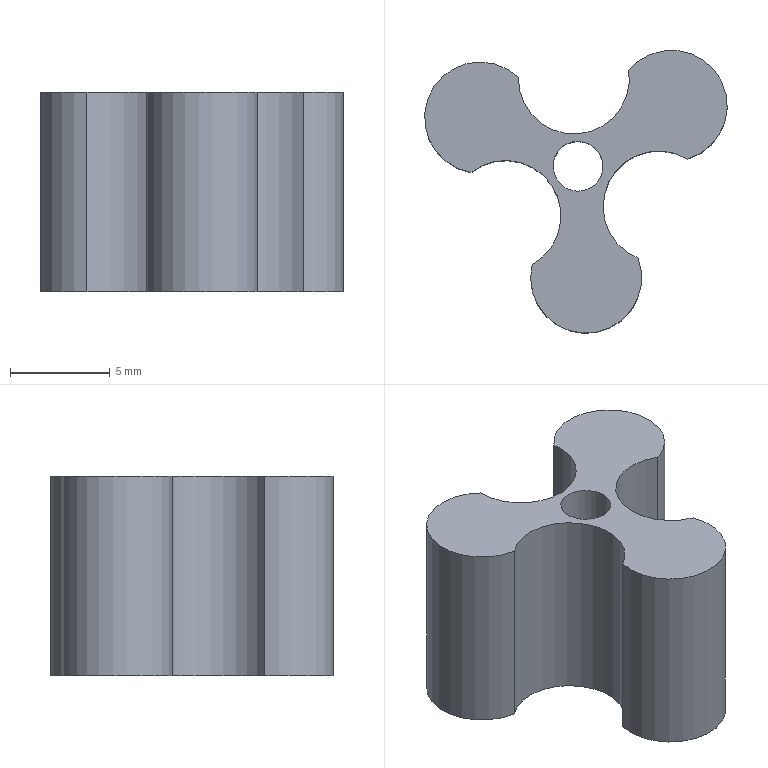Component | NX | ROTOR_2 | 1 solid | 9 faces | box 15.17 x 14.18 x 10 mm | volume 814 mm3 | cylinder 7 | plane 2 | commonest cylinder face diameters 5.568 x6 2.5 x1
STEP:
#1=CARTESIAN_POINT('',(0.,0.,0.));
#2=DIRECTION('',(0.,0.,1.));
#3=DIRECTION('',(1.,0.,0.));
#4=AXIS2_PLACEMENT_3D('',#1,#2,#3);
#5=CARTESIAN_POINT('',(8.277,-4.62,-5.));
#6=VERTEX_POINT('',#5);
#7=CARTESIAN_POINT('',(2.964,-4.947,-5.));
#8=VERTEX_POINT('',#7);
#9=CARTESIAN_POINT('',(5.671,-5.598,-5.));
#10=DIRECTION('',(0.,0.,-1.));
#11=DIRECTION('',(-0.06144,0.9981,0.));
#12=AXIS2_PLACEMENT_3D('',#9,#10,#11);
#13=CIRCLE('',#12,2.784);
#14=CARTESIAN_POINT('',(3.648,-4.052,-5.));
#15=DIRECTION('',(0.,0.,-1.));
#16=DIRECTION('',(-0.8337,-0.5523,0.));
#17=AXIS2_PLACEMENT_3D('',#14,#15,#16);
#18=PLANE('',#17);
#19=CARTESIAN_POINT('',(-0.833,-2.406));
#20=DIRECTION('',(-0.5,0.866));
#21=AXIS2_PLACEMENT_2D('',#19,#20);
#22=CIRCLE('',#21,2.784);
#23=(GEOMETRIC_REPRESENTATION_CONTEXT(2)PARAMETRIC_REPRESENTATION_CONTEXT()REPRESENTATION_CONTEXT('',''));
#24=DEFINITIONAL_REPRESENTATION('',(#22),#23);
#25=PCURVE('',#18,#24);
#26=CARTESIAN_POINT('',(5.671,-5.598,-5.));
#27=DIRECTION('',(0.,0.,1.));
#28=DIRECTION('',(0.8337,0.5523,0.));
#29=AXIS2_PLACEMENT_3D('',#26,#27,#28);
#30=CYLINDRICAL_SURFACE('',#29,2.784);
#31=CARTESIAN_POINT('',(7.33,0.));
#32=DIRECTION('',(-1.,0.));
#33=VECTOR('',#32,1.);
#34=LINE('',#31,#33);
#35=(GEOMETRIC_REPRESENTATION_CONTEXT(2)PARAMETRIC_REPRESENTATION_CONTEXT()REPRESENTATION_CONTEXT('',''));
#36=DEFINITIONAL_REPRESENTATION('',(#34),#35);
#37=PCURVE('',#30,#36);
#38=SURFACE_CURVE('',#13,(#25,#37),.PCURVE_S1.);
#39=EDGE_CURVE('',#6,#8,#38,.T.);
#40=ORIENTED_EDGE('',*,*,#39,.T.);
#41=CARTESIAN_POINT('',(-0.1006,-0.3217,-5.));
#42=VERTEX_POINT('',#41);
#43=CARTESIAN_POINT('',(1.625,-2.507,-5.));
#44=DIRECTION('',(0.,0.,1.));
#45=DIRECTION('',(-0.06144,0.9981,0.));
#46=AXIS2_PLACEMENT_3D('',#43,#44,#45);
#47=CIRCLE('',#46,2.784);
#48=CARTESIAN_POINT('',(-0.559,4.817));
#49=CARTESIAN_POINT('',(3.617,7.228));
#50=CARTESIAN_POINT('',(3.617,2.406));
#51=CARTESIAN_POINT('',(3.617,-2.416));
#52=CARTESIAN_POINT('',(-0.559,-0.005196));
#53=CARTESIAN_POINT('',(-4.735,2.406));
#54=CARTESIAN_POINT('',(-0.559,4.817));
#55=(BOUNDED_CURVE()B_SPLINE_CURVE(2,(#48,#49,#50,#51,#52,#53,#54),.UNSPECIFIED.,.T.,.F.)B_SPLINE_CURVE_WITH_KNOTS((1,2,2,2,2,1),(-2.094,0.,2.094,4.189,6.283,8.378),.UNSPECIFIED.)CURVE()GEOMETRIC_REPRESENTATION_ITEM()RATIONAL_B_SPLINE_CURVE((1.,0.5,1.,0.5,1.,0.5,1.))REPRESENTATION_ITEM(''));
#56=(GEOMETRIC_REPRESENTATION_CONTEXT(2)PARAMETRIC_REPRESENTATION_CONTEXT()REPRESENTATION_CONTEXT('',''));
#57=DEFINITIONAL_REPRESENTATION('',(#55),#56);
#58=PCURVE('',#18,#57);
#59=CARTESIAN_POINT('',(1.625,-2.507,-5.));
#60=DIRECTION('',(0.,0.,1.));
#61=DIRECTION('',(0.8337,0.5523,0.));
#62=AXIS2_PLACEMENT_3D('',#59,#60,#61);
#63=CYLINDRICAL_SURFACE('',#62,2.784);
#64=CARTESIAN_POINT('',(-5.236,0.));
#65=DIRECTION('',(1.,0.));
#66=VECTOR('',#65,1.);
#67=LINE('',#64,#66);
#68=(GEOMETRIC_REPRESENTATION_CONTEXT(2)PARAMETRIC_REPRESENTATION_CONTEXT()REPRESENTATION_CONTEXT('',''));
#69=DEFINITIONAL_REPRESENTATION('',(#67),#68);
#70=PCURVE('',#63,#69);
#71=SURFACE_CURVE('',#47,(#58,#70),.PCURVE_S1.);
#72=EDGE_CURVE('',#8,#42,#71,.T.);
#73=ORIENTED_EDGE('',*,*,#72,.T.);
#74=CARTESIAN_POINT('',(2.273,4.444,-5.));
#75=VERTEX_POINT('',#74);
#76=CARTESIAN_POINT('',(0.3561,2.425,-5.));
#77=DIRECTION('',(0.,0.,-1.));
#78=DIRECTION('',(-0.8337,-0.5523,0.));
#79=AXIS2_PLACEMENT_3D('',#76,#77,#78);
#80=CIRCLE('',#79,2.784);
#81=CARTESIAN_POINT('',(-0.833,7.217));
#82=DIRECTION('',(1.,0.));
#83=AXIS2_PLACEMENT_2D('',#81,#82);
#84=CIRCLE('',#83,2.784);
#85=(GEOMETRIC_REPRESENTATION_CONTEXT(2)PARAMETRIC_REPRESENTATION_CONTEXT()REPRESENTATION_CONTEXT('',''));
#86=DEFINITIONAL_REPRESENTATION('',(#84),#85);
#87=PCURVE('',#18,#86);
#88=CARTESIAN_POINT('',(0.3561,2.425,-5.));
#89=DIRECTION('',(0.,0.,1.));
#90=DIRECTION('',(0.8337,0.5523,0.));
#91=AXIS2_PLACEMENT_3D('',#88,#89,#90);
#92=CYLINDRICAL_SURFACE('',#91,2.784);
#93=CARTESIAN_POINT('',(9.425,0.));
#94=DIRECTION('',(-1.,0.));
#95=VECTOR('',#94,1.);
#96=LINE('',#93,#95);
#97=(GEOMETRIC_REPRESENTATION_CONTEXT(2)PARAMETRIC_REPRESENTATION_CONTEXT()REPRESENTATION_CONTEXT('',''));
#98=DEFINITIONAL_REPRESENTATION('',(#96),#97);
#99=PCURVE('',#92,#98);
#100=SURFACE_CURVE('',#80,(#87,#99),.PCURVE_S1.);
#101=EDGE_CURVE('',#42,#75,#100,.T.);
#102=ORIENTED_EDGE('',*,*,#101,.T.);
#103=CARTESIAN_POINT('',(7.811,4.785,-5.));
#104=VERTEX_POINT('',#103);
#105=CARTESIAN_POINT('',(5.056,4.383,-5.));
#106=DIRECTION('',(0.,0.,1.));
#107=DIRECTION('',(-0.06144,0.9981,0.));
#108=AXIS2_PLACEMENT_3D('',#105,#106,#107);
#109=CIRCLE('',#108,2.784);
#110=CARTESIAN_POINT('',(-7.225,8.665));
#111=CARTESIAN_POINT('',(-3.049,11.076));
#112=CARTESIAN_POINT('',(-3.049,6.254));
#113=CARTESIAN_POINT('',(-3.049,1.432));
#114=CARTESIAN_POINT('',(-7.225,3.843));
#115=CARTESIAN_POINT('',(-11.401,6.254));
#116=CARTESIAN_POINT('',(-7.225,8.665));
#117=(BOUNDED_CURVE()B_SPLINE_CURVE(2,(#110,#111,#112,#113,#114,#115,#116),.UNSPECIFIED.,.T.,.F.)B_SPLINE_CURVE_WITH_KNOTS((1,2,2,2,2,1),(-2.094,0.,2.094,4.189,6.283,8.378),.UNSPECIFIED.)CURVE()GEOMETRIC_REPRESENTATION_ITEM()RATIONAL_B_SPLINE_CURVE((1.,0.5,1.,0.5,1.,0.5,1.))REPRESENTATION_ITEM(''));
#118=(GEOMETRIC_REPRESENTATION_CONTEXT(2)PARAMETRIC_REPRESENTATION_CONTEXT()REPRESENTATION_CONTEXT('',''));
#119=DEFINITIONAL_REPRESENTATION('',(#117),#118);
#120=PCURVE('',#18,#119);
#121=CARTESIAN_POINT('',(5.056,4.383,-5.));
#122=DIRECTION('',(0.,0.,1.));
#123=DIRECTION('',(0.8337,0.5523,0.));
#124=AXIS2_PLACEMENT_3D('',#121,#122,#123);
#125=CYLINDRICAL_SURFACE('',#124,2.784);
#126=CARTESIAN_POINT('',(1.047,0.));
#127=DIRECTION('',(1.,0.));
#128=VECTOR('',#127,1.);
#129=LINE('',#126,#128);
#130=(GEOMETRIC_REPRESENTATION_CONTEXT(2)PARAMETRIC_REPRESENTATION_CONTEXT()REPRESENTATION_CONTEXT('',''));
#131=DEFINITIONAL_REPRESENTATION('',(#129),#130);
#132=PCURVE('',#125,#131);
#133=SURFACE_CURVE('',#109,(#120,#132),.PCURVE_S1.);
#134=EDGE_CURVE('',#75,#104,#133,.T.);
#135=ORIENTED_EDGE('',*,*,#134,.T.);
#136=CARTESIAN_POINT('',(10.751,0.3464,-5.));
#137=VERTEX_POINT('',#136);
#138=CARTESIAN_POINT('',(9.961,3.016,-5.));
#139=DIRECTION('',(0.,0.,-1.));
#140=DIRECTION('',(-0.8337,-0.5523,0.));
#141=AXIS2_PLACEMENT_3D('',#138,#139,#140);
#142=CIRCLE('',#141,2.784);
#143=CARTESIAN_POINT('',(-9.167,2.406));
#144=DIRECTION('',(1.,0.));
#145=AXIS2_PLACEMENT_2D('',#143,#144);
#146=CIRCLE('',#145,2.784);
#147=(GEOMETRIC_REPRESENTATION_CONTEXT(2)PARAMETRIC_REPRESENTATION_CONTEXT()REPRESENTATION_CONTEXT('',''));
#148=DEFINITIONAL_REPRESENTATION('',(#146),#147);
#149=PCURVE('',#18,#148);
#150=CARTESIAN_POINT('',(9.961,3.016,-5.));
#151=DIRECTION('',(0.,0.,1.));
#152=DIRECTION('',(0.8337,0.5523,0.));
#153=AXIS2_PLACEMENT_3D('',#150,#151,#152);
#154=CYLINDRICAL_SURFACE('',#153,2.784);
#155=CARTESIAN_POINT('',(9.425,0.));
#156=DIRECTION('',(-1.,0.));
#157=VECTOR('',#156,1.);
#158=LINE('',#155,#157);
#159=(GEOMETRIC_REPRESENTATION_CONTEXT(2)PARAMETRIC_REPRESENTATION_CONTEXT()REPRESENTATION_CONTEXT('',''));
#160=DEFINITIONAL_REPRESENTATION('',(#158),#159);
#161=PCURVE('',#154,#160);
#162=SURFACE_CURVE('',#142,(#149,#161),.PCURVE_S1.);
#163=EDGE_CURVE('',#104,#137,#162,.T.);
#164=ORIENTED_EDGE('',*,*,#163,.T.);
#165=CARTESIAN_POINT('',(9.307,-2.034,-5.));
#166=DIRECTION('',(0.,0.,1.));
#167=DIRECTION('',(-0.06144,0.9981,0.));
#168=AXIS2_PLACEMENT_3D('',#165,#166,#167);
#169=CIRCLE('',#168,2.784);
#170=CARTESIAN_POINT('',(-7.225,0.9682));
#171=CARTESIAN_POINT('',(-3.049,3.379));
#172=CARTESIAN_POINT('',(-3.049,-1.443));
#173=CARTESIAN_POINT('',(-3.049,-6.265));
#174=CARTESIAN_POINT('',(-7.225,-3.854));
#175=CARTESIAN_POINT('',(-11.401,-1.443));
#176=CARTESIAN_POINT('',(-7.225,0.9682));
#177=(BOUNDED_CURVE()B_SPLINE_CURVE(2,(#170,#171,#172,#173,#174,#175,#176),.UNSPECIFIED.,.T.,.F.)B_SPLINE_CURVE_WITH_KNOTS((1,2,2,2,2,1),(-2.094,0.,2.094,4.189,6.283,8.378),.UNSPECIFIED.)CURVE()GEOMETRIC_REPRESENTATION_ITEM()RATIONAL_B_SPLINE_CURVE((1.,0.5,1.,0.5,1.,0.5,1.))REPRESENTATION_ITEM(''));
#178=(GEOMETRIC_REPRESENTATION_CONTEXT(2)PARAMETRIC_REPRESENTATION_CONTEXT()REPRESENTATION_CONTEXT('',''));
#179=DEFINITIONAL_REPRESENTATION('',(#177),#178);
#180=PCURVE('',#18,#179);
#181=CARTESIAN_POINT('',(9.307,-2.034,-5.));
#182=DIRECTION('',(0.,0.,1.));
#183=DIRECTION('',(0.8337,0.5523,0.));
#184=AXIS2_PLACEMENT_3D('',#181,#182,#183);
#185=CYLINDRICAL_SURFACE('',#184,2.784);
#186=CARTESIAN_POINT('',(-5.236,0.));
#187=DIRECTION('',(1.,0.));
#188=VECTOR('',#187,1.);
#189=LINE('',#186,#188);
#190=(GEOMETRIC_REPRESENTATION_CONTEXT(2)PARAMETRIC_REPRESENTATION_CONTEXT()REPRESENTATION_CONTEXT('',''));
#191=DEFINITIONAL_REPRESENTATION('',(#189),#190);
#192=PCURVE('',#185,#191);
#193=SURFACE_CURVE('',#169,(#180,#192),.PCURVE_S1.);
#194=EDGE_CURVE('',#137,#6,#193,.T.);
#195=ORIENTED_EDGE('',*,*,#194,.T.);
#196=EDGE_LOOP('',(#40,#73,#102,#135,#164,#195));
#197=FACE_BOUND('',#196,.T.);
#198=CARTESIAN_POINT('',(4.224,-0.7066,-5.));
#199=VERTEX_POINT('',#198);
#200=CARTESIAN_POINT('',(5.266,-0.01624,-5.));
#201=DIRECTION('',(0.,0.,1.));
#202=DIRECTION('',(-0.8337,-0.5523,0.));
#203=AXIS2_PLACEMENT_3D('',#200,#201,#202);
#204=CIRCLE('',#203,1.25);
#205=CARTESIAN_POINT('',(-2.328,2.471));
#206=CARTESIAN_POINT('',(-2.328,0.3058));
#207=CARTESIAN_POINT('',(-4.203,1.388));
#208=CARTESIAN_POINT('',(-6.078,2.471));
#209=CARTESIAN_POINT('',(-4.203,3.553));
#210=CARTESIAN_POINT('',(-2.328,4.636));
#211=CARTESIAN_POINT('',(-2.328,2.471));
#212=(BOUNDED_CURVE()B_SPLINE_CURVE(2,(#205,#206,#207,#208,#209,#210,#211),.UNSPECIFIED.,.T.,.F.)B_SPLINE_CURVE_WITH_KNOTS((1,2,2,2,2,1),(-2.094,0.,2.094,4.189,6.283,8.378),.UNSPECIFIED.)CURVE()GEOMETRIC_REPRESENTATION_ITEM()RATIONAL_B_SPLINE_CURVE((1.,0.5,1.,0.5,1.,0.5,1.))REPRESENTATION_ITEM(''));
#213=(GEOMETRIC_REPRESENTATION_CONTEXT(2)PARAMETRIC_REPRESENTATION_CONTEXT()REPRESENTATION_CONTEXT('',''));
#214=DEFINITIONAL_REPRESENTATION('',(#212),#213);
#215=PCURVE('',#18,#214);
#216=CARTESIAN_POINT('',(5.266,-0.01624,-7.));
#217=DIRECTION('',(0.,0.,1.));
#218=DIRECTION('',(0.8337,0.5523,0.));
#219=AXIS2_PLACEMENT_3D('',#216,#217,#218);
#220=CYLINDRICAL_SURFACE('',#219,1.25);
#221=CARTESIAN_POINT('',(3.142,2.));
#222=DIRECTION('',(1.,0.));
#223=VECTOR('',#222,1.);
#224=LINE('',#221,#223);
#225=(GEOMETRIC_REPRESENTATION_CONTEXT(2)PARAMETRIC_REPRESENTATION_CONTEXT()REPRESENTATION_CONTEXT('',''));
#226=DEFINITIONAL_REPRESENTATION('',(#224),#225);
#227=PCURVE('',#220,#226);
#228=SURFACE_CURVE('',#204,(#215,#227),.PCURVE_S1.);
#229=EDGE_CURVE('',#199,#199,#228,.T.);
#230=ORIENTED_EDGE('',*,*,#229,.T.);
#231=EDGE_LOOP('',(#230));
#232=FACE_BOUND('',#231,.T.);
#233=ADVANCED_FACE('',(#197,#232),#18,.T.);
#234=CARTESIAN_POINT('',(2.964,-4.947,5.));
#235=VERTEX_POINT('',#234);
#236=CARTESIAN_POINT('',(-0.1006,-0.3217,5.));
#237=VERTEX_POINT('',#236);
#238=CARTESIAN_POINT('',(1.625,-2.507,5.));
#239=DIRECTION('',(0.,0.,1.));
#240=DIRECTION('',(-0.8337,-0.5523,0.));
#241=AXIS2_PLACEMENT_3D('',#238,#239,#240);
#242=CIRCLE('',#241,2.784);
#243=CARTESIAN_POINT('',(3.648,-4.052,5.));
#244=DIRECTION('',(0.,0.,-1.));
#245=DIRECTION('',(-0.8337,-0.5523,0.));
#246=AXIS2_PLACEMENT_3D('',#243,#244,#245);
#247=PLANE('',#246);
#248=CARTESIAN_POINT('',(3.617,2.406));
#249=CARTESIAN_POINT('',(3.617,-2.416));
#250=CARTESIAN_POINT('',(-0.559,-0.005196));
#251=CARTESIAN_POINT('',(-4.735,2.406));
#252=CARTESIAN_POINT('',(-0.559,4.817));
#253=CARTESIAN_POINT('',(3.617,7.228));
#254=CARTESIAN_POINT('',(3.617,2.406));
#255=(BOUNDED_CURVE()B_SPLINE_CURVE(2,(#248,#249,#250,#251,#252,#253,#254),.UNSPECIFIED.,.T.,.F.)B_SPLINE_CURVE_WITH_KNOTS((1,2,2,2,2,1),(-2.094,0.,2.094,4.189,6.283,8.378),.UNSPECIFIED.)CURVE()GEOMETRIC_REPRESENTATION_ITEM()RATIONAL_B_SPLINE_CURVE((1.,0.5,1.,0.5,1.,0.5,1.))REPRESENTATION_ITEM(''));
#256=(GEOMETRIC_REPRESENTATION_CONTEXT(2)PARAMETRIC_REPRESENTATION_CONTEXT()REPRESENTATION_CONTEXT('',''));
#257=DEFINITIONAL_REPRESENTATION('',(#255),#256);
#258=PCURVE('',#247,#257);
#259=CARTESIAN_POINT('',(-3.142,10.));
#260=DIRECTION('',(1.,0.));
#261=VECTOR('',#260,1.);
#262=LINE('',#259,#261);
#263=(GEOMETRIC_REPRESENTATION_CONTEXT(2)PARAMETRIC_REPRESENTATION_CONTEXT()REPRESENTATION_CONTEXT('',''));
#264=DEFINITIONAL_REPRESENTATION('',(#262),#263);
#265=PCURVE('',#63,#264);
#266=SURFACE_CURVE('',#242,(#258,#265),.PCURVE_S1.);
#267=EDGE_CURVE('',#235,#237,#266,.T.);
#268=ORIENTED_EDGE('',*,*,#267,.F.);
#269=CARTESIAN_POINT('',(8.277,-4.62,5.));
#270=VERTEX_POINT('',#269);
#271=CARTESIAN_POINT('',(5.671,-5.598,5.));
#272=DIRECTION('',(0.,0.,-1.));
#273=DIRECTION('',(-0.8337,-0.5523,0.));
#274=AXIS2_PLACEMENT_3D('',#271,#272,#273);
#275=CIRCLE('',#274,2.784);
#276=CARTESIAN_POINT('',(-0.833,-2.406));
#277=DIRECTION('',(1.,0.));
#278=AXIS2_PLACEMENT_2D('',#276,#277);
#279=CIRCLE('',#278,2.784);
#280=(GEOMETRIC_REPRESENTATION_CONTEXT(2)PARAMETRIC_REPRESENTATION_CONTEXT()REPRESENTATION_CONTEXT('',''));
#281=DEFINITIONAL_REPRESENTATION('',(#279),#280);
#282=PCURVE('',#247,#281);
#283=CARTESIAN_POINT('',(9.425,10.));
#284=DIRECTION('',(-1.,0.));
#285=VECTOR('',#284,1.);
#286=LINE('',#283,#285);
#287=(GEOMETRIC_REPRESENTATION_CONTEXT(2)PARAMETRIC_REPRESENTATION_CONTEXT()REPRESENTATION_CONTEXT('',''));
#288=DEFINITIONAL_REPRESENTATION('',(#286),#287);
#289=PCURVE('',#30,#288);
#290=SURFACE_CURVE('',#275,(#282,#289),.PCURVE_S1.);
#291=EDGE_CURVE('',#270,#235,#290,.T.);
#292=ORIENTED_EDGE('',*,*,#291,.F.);
#293=CARTESIAN_POINT('',(10.751,0.3464,5.));
#294=VERTEX_POINT('',#293);
#295=CARTESIAN_POINT('',(9.307,-2.034,5.));
#296=DIRECTION('',(0.,0.,1.));
#297=DIRECTION('',(-0.8337,-0.5523,0.));
#298=AXIS2_PLACEMENT_3D('',#295,#296,#297);
#299=CIRCLE('',#298,2.784);
#300=CARTESIAN_POINT('',(-3.049,-1.443));
#301=CARTESIAN_POINT('',(-3.049,-6.265));
#302=CARTESIAN_POINT('',(-7.225,-3.854));
#303=CARTESIAN_POINT('',(-11.401,-1.443));
#304=CARTESIAN_POINT('',(-7.225,0.9682));
#305=CARTESIAN_POINT('',(-3.049,3.379));
#306=CARTESIAN_POINT('',(-3.049,-1.443));
#307=(BOUNDED_CURVE()B_SPLINE_CURVE(2,(#300,#301,#302,#303,#304,#305,#306),.UNSPECIFIED.,.T.,.F.)B_SPLINE_CURVE_WITH_KNOTS((1,2,2,2,2,1),(-2.094,0.,2.094,4.189,6.283,8.378),.UNSPECIFIED.)CURVE()GEOMETRIC_REPRESENTATION_ITEM()RATIONAL_B_SPLINE_CURVE((1.,0.5,1.,0.5,1.,0.5,1.))REPRESENTATION_ITEM(''));
#308=(GEOMETRIC_REPRESENTATION_CONTEXT(2)PARAMETRIC_REPRESENTATION_CONTEXT()REPRESENTATION_CONTEXT('',''));
#309=DEFINITIONAL_REPRESENTATION('',(#307),#308);
#310=PCURVE('',#247,#309);
#311=CARTESIAN_POINT('',(-3.142,10.));
#312=DIRECTION('',(1.,0.));
#313=VECTOR('',#312,1.);
#314=LINE('',#311,#313);
#315=(GEOMETRIC_REPRESENTATION_CONTEXT(2)PARAMETRIC_REPRESENTATION_CONTEXT()REPRESENTATION_CONTEXT('',''));
#316=DEFINITIONAL_REPRESENTATION('',(#314),#315);
#317=PCURVE('',#185,#316);
#318=SURFACE_CURVE('',#299,(#310,#317),.PCURVE_S1.);
#319=EDGE_CURVE('',#294,#270,#318,.T.);
#320=ORIENTED_EDGE('',*,*,#319,.F.);
#321=CARTESIAN_POINT('',(7.811,4.785,5.));
#322=VERTEX_POINT('',#321);
#323=CARTESIAN_POINT('',(9.961,3.016,5.));
#324=DIRECTION('',(0.,0.,-1.));
#325=DIRECTION('',(-0.06144,0.9981,0.));
#326=AXIS2_PLACEMENT_3D('',#323,#324,#325);
#327=CIRCLE('',#326,2.784);
#328=CARTESIAN_POINT('',(-9.167,2.406));
#329=DIRECTION('',(-0.5,0.866));
#330=AXIS2_PLACEMENT_2D('',#328,#329);
#331=CIRCLE('',#330,2.784);
#332=(GEOMETRIC_REPRESENTATION_CONTEXT(2)PARAMETRIC_REPRESENTATION_CONTEXT()REPRESENTATION_CONTEXT('',''));
#333=DEFINITIONAL_REPRESENTATION('',(#331),#332);
#334=PCURVE('',#247,#333);
#335=CARTESIAN_POINT('',(13.614,10.));
#336=DIRECTION('',(-1.,0.));
#337=VECTOR('',#336,1.);
#338=LINE('',#335,#337);
#339=(GEOMETRIC_REPRESENTATION_CONTEXT(2)PARAMETRIC_REPRESENTATION_CONTEXT()REPRESENTATION_CONTEXT('',''));
#340=DEFINITIONAL_REPRESENTATION('',(#338),#339);
#341=PCURVE('',#154,#340);
#342=SURFACE_CURVE('',#327,(#334,#341),.PCURVE_S1.);
#343=EDGE_CURVE('',#322,#294,#342,.T.);
#344=ORIENTED_EDGE('',*,*,#343,.F.);
#345=CARTESIAN_POINT('',(2.273,4.444,5.));
#346=VERTEX_POINT('',#345);
#347=CARTESIAN_POINT('',(5.056,4.383,5.));
#348=DIRECTION('',(0.,0.,1.));
#349=DIRECTION('',(-0.8337,-0.5523,0.));
#350=AXIS2_PLACEMENT_3D('',#347,#348,#349);
#351=CIRCLE('',#350,2.784);
#352=CARTESIAN_POINT('',(-3.049,6.254));
#353=CARTESIAN_POINT('',(-3.049,1.432));
#354=CARTESIAN_POINT('',(-7.225,3.843));
#355=CARTESIAN_POINT('',(-11.401,6.254));
#356=CARTESIAN_POINT('',(-7.225,8.665));
#357=CARTESIAN_POINT('',(-3.049,11.076));
#358=CARTESIAN_POINT('',(-3.049,6.254));
#359=(BOUNDED_CURVE()B_SPLINE_CURVE(2,(#352,#353,#354,#355,#356,#357,#358),.UNSPECIFIED.,.T.,.F.)B_SPLINE_CURVE_WITH_KNOTS((1,2,2,2,2,1),(-2.094,0.,2.094,4.189,6.283,8.378),.UNSPECIFIED.)CURVE()GEOMETRIC_REPRESENTATION_ITEM()RATIONAL_B_SPLINE_CURVE((1.,0.5,1.,0.5,1.,0.5,1.))REPRESENTATION_ITEM(''));
#360=(GEOMETRIC_REPRESENTATION_CONTEXT(2)PARAMETRIC_REPRESENTATION_CONTEXT()REPRESENTATION_CONTEXT('',''));
#361=DEFINITIONAL_REPRESENTATION('',(#359),#360);
#362=PCURVE('',#247,#361);
#363=CARTESIAN_POINT('',(-3.142,10.));
#364=DIRECTION('',(1.,0.));
#365=VECTOR('',#364,1.);
#366=LINE('',#363,#365);
#367=(GEOMETRIC_REPRESENTATION_CONTEXT(2)PARAMETRIC_REPRESENTATION_CONTEXT()REPRESENTATION_CONTEXT('',''));
#368=DEFINITIONAL_REPRESENTATION('',(#366),#367);
#369=PCURVE('',#125,#368);
#370=SURFACE_CURVE('',#351,(#362,#369),.PCURVE_S1.);
#371=EDGE_CURVE('',#346,#322,#370,.T.);
#372=ORIENTED_EDGE('',*,*,#371,.F.);
#373=CARTESIAN_POINT('',(0.3561,2.425,5.));
#374=DIRECTION('',(0.,0.,-1.));
#375=DIRECTION('',(-0.06144,0.9981,0.));
#376=AXIS2_PLACEMENT_3D('',#373,#374,#375);
#377=CIRCLE('',#376,2.784);
#378=CARTESIAN_POINT('',(-0.833,7.217));
#379=DIRECTION('',(-0.5,0.866));
#380=AXIS2_PLACEMENT_2D('',#378,#379);
#381=CIRCLE('',#380,2.784);
#382=(GEOMETRIC_REPRESENTATION_CONTEXT(2)PARAMETRIC_REPRESENTATION_CONTEXT()REPRESENTATION_CONTEXT('',''));
#383=DEFINITIONAL_REPRESENTATION('',(#381),#382);
#384=PCURVE('',#247,#383);
#385=CARTESIAN_POINT('',(7.33,10.));
#386=DIRECTION('',(-1.,0.));
#387=VECTOR('',#386,1.);
#388=LINE('',#385,#387);
#389=(GEOMETRIC_REPRESENTATION_CONTEXT(2)PARAMETRIC_REPRESENTATION_CONTEXT()REPRESENTATION_CONTEXT('',''));
#390=DEFINITIONAL_REPRESENTATION('',(#388),#389);
#391=PCURVE('',#92,#390);
#392=SURFACE_CURVE('',#377,(#384,#391),.PCURVE_S1.);
#393=EDGE_CURVE('',#237,#346,#392,.T.);
#394=ORIENTED_EDGE('',*,*,#393,.F.);
#395=EDGE_LOOP('',(#268,#292,#320,#344,#372,#394));
#396=FACE_BOUND('',#395,.T.);
#397=CARTESIAN_POINT('',(4.224,-0.7066,5.));
#398=VERTEX_POINT('',#397);
#399=CARTESIAN_POINT('',(5.266,-0.01624,5.));
#400=DIRECTION('',(0.,0.,-1.));
#401=DIRECTION('',(-0.8337,-0.5523,0.));
#402=AXIS2_PLACEMENT_3D('',#399,#400,#401);
#403=CIRCLE('',#402,1.25);
#404=CARTESIAN_POINT('',(-3.578,2.471));
#405=DIRECTION('',(1.,0.));
#406=AXIS2_PLACEMENT_2D('',#404,#405);
#407=CIRCLE('',#406,1.25);
#408=(GEOMETRIC_REPRESENTATION_CONTEXT(2)PARAMETRIC_REPRESENTATION_CONTEXT()REPRESENTATION_CONTEXT('',''));
#409=DEFINITIONAL_REPRESENTATION('',(#407),#408);
#410=PCURVE('',#247,#409);
#411=CARTESIAN_POINT('',(9.425,12.));
#412=DIRECTION('',(-1.,0.));
#413=VECTOR('',#412,1.);
#414=LINE('',#411,#413);
#415=(GEOMETRIC_REPRESENTATION_CONTEXT(2)PARAMETRIC_REPRESENTATION_CONTEXT()REPRESENTATION_CONTEXT('',''));
#416=DEFINITIONAL_REPRESENTATION('',(#414),#415);
#417=PCURVE('',#220,#416);
#418=SURFACE_CURVE('',#403,(#410,#417),.PCURVE_S1.);
#419=EDGE_CURVE('',#398,#398,#418,.T.);
#420=ORIENTED_EDGE('',*,*,#419,.T.);
#421=EDGE_LOOP('',(#420));
#422=FACE_BOUND('',#421,.T.);
#423=ADVANCED_FACE('',(#396,#422),#247,.F.);
#424=CARTESIAN_POINT('',(2.964,-4.947,-5.));
#425=DIRECTION('',(0.,0.,1.));
#426=VECTOR('',#425,1.);
#427=LINE('',#424,#426);
#428=CARTESIAN_POINT('',(-1.654,0.));
#429=DIRECTION('',(0.,1.));
#430=VECTOR('',#429,1.);
#431=LINE('',#428,#430);
#432=(GEOMETRIC_REPRESENTATION_CONTEXT(2)PARAMETRIC_REPRESENTATION_CONTEXT()REPRESENTATION_CONTEXT('',''));
#433=DEFINITIONAL_REPRESENTATION('',(#431),#432);
#434=PCURVE('',#63,#433);
#435=CARTESIAN_POINT('',(2.321,0.));
#436=DIRECTION('',(0.,1.));
#437=VECTOR('',#436,1.);
#438=LINE('',#435,#437);
#439=(GEOMETRIC_REPRESENTATION_CONTEXT(2)PARAMETRIC_REPRESENTATION_CONTEXT()REPRESENTATION_CONTEXT('',''));
#440=DEFINITIONAL_REPRESENTATION('',(#438),#439);
#441=PCURVE('',#30,#440);
#442=SURFACE_CURVE('',#427,(#434,#441),.PCURVE_S1.);
#443=EDGE_CURVE('',#8,#235,#442,.T.);
#444=ORIENTED_EDGE('',*,*,#443,.F.);
#445=ORIENTED_EDGE('',*,*,#72,.T.);
#446=CARTESIAN_POINT('',(-0.1006,-0.3217,-5.));
#447=DIRECTION('',(0.,0.,1.));
#448=VECTOR('',#447,1.);
#449=LINE('',#446,#448);
#450=CARTESIAN_POINT('',(1.654,0.));
#451=DIRECTION('',(0.,1.));
#452=VECTOR('',#451,1.);
#453=LINE('',#450,#452);
#454=(GEOMETRIC_REPRESENTATION_CONTEXT(2)PARAMETRIC_REPRESENTATION_CONTEXT()REPRESENTATION_CONTEXT('',''));
#455=DEFINITIONAL_REPRESENTATION('',(#453),#454);
#456=PCURVE('',#63,#455);
#457=CARTESIAN_POINT('',(3.963,0.));
#458=DIRECTION('',(0.,1.));
#459=VECTOR('',#458,1.);
#460=LINE('',#457,#459);
#461=(GEOMETRIC_REPRESENTATION_CONTEXT(2)PARAMETRIC_REPRESENTATION_CONTEXT()REPRESENTATION_CONTEXT('',''));
#462=DEFINITIONAL_REPRESENTATION('',(#460),#461);
#463=PCURVE('',#92,#462);
#464=SURFACE_CURVE('',#449,(#456,#463),.PCURVE_S1.);
#465=EDGE_CURVE('',#42,#237,#464,.T.);
#466=ORIENTED_EDGE('',*,*,#465,.T.);
#467=ORIENTED_EDGE('',*,*,#267,.F.);
#468=EDGE_LOOP('',(#444,#445,#466,#467));
#469=FACE_BOUND('',#468,.F.);
#470=ADVANCED_FACE('',(#469),#63,.F.);
#471=ORIENTED_EDGE('',*,*,#393,.T.);
#472=CARTESIAN_POINT('',(2.273,4.444,-5.));
#473=DIRECTION('',(0.,0.,1.));
#474=VECTOR('',#473,1.);
#475=LINE('',#472,#474);
#476=CARTESIAN_POINT('',(0.2263,0.));
#477=DIRECTION('',(0.,1.));
#478=VECTOR('',#477,1.);
#479=LINE('',#476,#478);
#480=(GEOMETRIC_REPRESENTATION_CONTEXT(2)PARAMETRIC_REPRESENTATION_CONTEXT()REPRESENTATION_CONTEXT('',''));
#481=DEFINITIONAL_REPRESENTATION('',(#479),#480);
#482=PCURVE('',#92,#481);
#483=CARTESIAN_POINT('',(2.535,0.));
#484=DIRECTION('',(0.,1.));
#485=VECTOR('',#484,1.);
#486=LINE('',#483,#485);
#487=(GEOMETRIC_REPRESENTATION_CONTEXT(2)PARAMETRIC_REPRESENTATION_CONTEXT()REPRESENTATION_CONTEXT('',''));
#488=DEFINITIONAL_REPRESENTATION('',(#486),#487);
#489=PCURVE('',#125,#488);
#490=SURFACE_CURVE('',#475,(#482,#489),.PCURVE_S1.);
#491=EDGE_CURVE('',#75,#346,#490,.T.);
#492=ORIENTED_EDGE('',*,*,#491,.F.);
#493=ORIENTED_EDGE('',*,*,#101,.F.);
#494=ORIENTED_EDGE('',*,*,#465,.T.);
#495=EDGE_LOOP('',(#471,#492,#493,#494));
#496=FACE_BOUND('',#495,.T.);
#497=ADVANCED_FACE('',(#496),#92,.T.);
#498=ORIENTED_EDGE('',*,*,#491,.F.);
#499=ORIENTED_EDGE('',*,*,#134,.T.);
#500=CARTESIAN_POINT('',(7.811,4.785,-5.));
#501=DIRECTION('',(0.,0.,1.));
#502=VECTOR('',#501,1.);
#503=LINE('',#500,#502);
#504=CARTESIAN_POINT('',(5.843,0.));
#505=DIRECTION('',(0.,1.));
#506=VECTOR('',#505,1.);
#507=LINE('',#504,#506);
#508=(GEOMETRIC_REPRESENTATION_CONTEXT(2)PARAMETRIC_REPRESENTATION_CONTEXT()REPRESENTATION_CONTEXT('',''));
#509=DEFINITIONAL_REPRESENTATION('',(#507),#508);
#510=PCURVE('',#125,#509);
#511=CARTESIAN_POINT('',(8.151,0.));
#512=DIRECTION('',(0.,1.));
#513=VECTOR('',#512,1.);
#514=LINE('',#511,#513);
#515=(GEOMETRIC_REPRESENTATION_CONTEXT(2)PARAMETRIC_REPRESENTATION_CONTEXT()REPRESENTATION_CONTEXT('',''));
#516=DEFINITIONAL_REPRESENTATION('',(#514),#515);
#517=PCURVE('',#154,#516);
#518=SURFACE_CURVE('',#503,(#510,#517),.PCURVE_S1.);
#519=EDGE_CURVE('',#104,#322,#518,.T.);
#520=ORIENTED_EDGE('',*,*,#519,.T.);
#521=ORIENTED_EDGE('',*,*,#371,.F.);
#522=EDGE_LOOP('',(#498,#499,#520,#521));
#523=FACE_BOUND('',#522,.F.);
#524=ADVANCED_FACE('',(#523),#125,.F.);
#525=ORIENTED_EDGE('',*,*,#343,.T.);
#526=CARTESIAN_POINT('',(10.751,0.3464,-5.));
#527=DIRECTION('',(0.,0.,1.));
#528=VECTOR('',#527,1.);
#529=LINE('',#526,#528);
#530=CARTESIAN_POINT('',(4.415,0.));
#531=DIRECTION('',(0.,1.));
#532=VECTOR('',#531,1.);
#533=LINE('',#530,#532);
#534=(GEOMETRIC_REPRESENTATION_CONTEXT(2)PARAMETRIC_REPRESENTATION_CONTEXT()REPRESENTATION_CONTEXT('',''));
#535=DEFINITIONAL_REPRESENTATION('',(#533),#534);
#536=PCURVE('',#154,#535);
#537=CARTESIAN_POINT('',(0.4404,0.));
#538=DIRECTION('',(0.,1.));
#539=VECTOR('',#538,1.);
#540=LINE('',#537,#539);
#541=(GEOMETRIC_REPRESENTATION_CONTEXT(2)PARAMETRIC_REPRESENTATION_CONTEXT()REPRESENTATION_CONTEXT('',''));
#542=DEFINITIONAL_REPRESENTATION('',(#540),#541);
#543=PCURVE('',#185,#542);
#544=SURFACE_CURVE('',#529,(#536,#543),.PCURVE_S1.);
#545=EDGE_CURVE('',#137,#294,#544,.T.);
#546=ORIENTED_EDGE('',*,*,#545,.F.);
#547=ORIENTED_EDGE('',*,*,#163,.F.);
#548=ORIENTED_EDGE('',*,*,#519,.T.);
#549=EDGE_LOOP('',(#525,#546,#547,#548));
#550=FACE_BOUND('',#549,.T.);
#551=ADVANCED_FACE('',(#550),#154,.T.);
#552=ORIENTED_EDGE('',*,*,#545,.F.);
#553=ORIENTED_EDGE('',*,*,#194,.T.);
#554=CARTESIAN_POINT('',(8.277,-4.62,-5.));
#555=DIRECTION('',(0.,0.,1.));
#556=VECTOR('',#555,1.);
#557=LINE('',#554,#556);
#558=CARTESIAN_POINT('',(3.748,0.));
#559=DIRECTION('',(0.,1.));
#560=VECTOR('',#559,1.);
#561=LINE('',#558,#560);
#562=(GEOMETRIC_REPRESENTATION_CONTEXT(2)PARAMETRIC_REPRESENTATION_CONTEXT()REPRESENTATION_CONTEXT('',''));
#563=DEFINITIONAL_REPRESENTATION('',(#561),#562);
#564=PCURVE('',#185,#563);
#565=CARTESIAN_POINT('',(6.057,0.));
#566=DIRECTION('',(0.,1.));
#567=VECTOR('',#566,1.);
#568=LINE('',#565,#567);
#569=(GEOMETRIC_REPRESENTATION_CONTEXT(2)PARAMETRIC_REPRESENTATION_CONTEXT()REPRESENTATION_CONTEXT('',''));
#570=DEFINITIONAL_REPRESENTATION('',(#568),#569);
#571=PCURVE('',#30,#570);
#572=SURFACE_CURVE('',#557,(#564,#571),.PCURVE_S1.);
#573=EDGE_CURVE('',#6,#270,#572,.T.);
#574=ORIENTED_EDGE('',*,*,#573,.T.);
#575=ORIENTED_EDGE('',*,*,#319,.F.);
#576=EDGE_LOOP('',(#552,#553,#574,#575));
#577=FACE_BOUND('',#576,.F.);
#578=ADVANCED_FACE('',(#577),#185,.F.);
#579=ORIENTED_EDGE('',*,*,#291,.T.);
#580=ORIENTED_EDGE('',*,*,#443,.F.);
#581=ORIENTED_EDGE('',*,*,#39,.F.);
#582=ORIENTED_EDGE('',*,*,#573,.T.);
#583=EDGE_LOOP('',(#579,#580,#581,#582));
#584=FACE_BOUND('',#583,.T.);
#585=ADVANCED_FACE('',(#584),#30,.T.);
#586=ORIENTED_EDGE('',*,*,#229,.T.);
#587=CARTESIAN_POINT('',(4.224,-0.7066,-5.));
#588=CARTESIAN_POINT('',(4.224,-0.7066,5.));
#589=B_SPLINE_CURVE_WITH_KNOTS('',1,(#587,#588),.UNSPECIFIED.,.F.,.F.,(2,2),(2.,12.),.PIECEWISE_BEZIER_KNOTS.);
#590=CARTESIAN_POINT('',(9.425,0.));
#591=DIRECTION('',(0.,1.));
#592=VECTOR('',#591,1.);
#593=LINE('',#590,#592);
#594=(GEOMETRIC_REPRESENTATION_CONTEXT(2)PARAMETRIC_REPRESENTATION_CONTEXT()REPRESENTATION_CONTEXT('',''));
#595=DEFINITIONAL_REPRESENTATION('',(#593),#594);
#596=PCURVE('',#220,#595);
#597=CARTESIAN_POINT('',(3.142,0.));
#598=DIRECTION('',(0.,1.));
#599=VECTOR('',#598,1.);
#600=LINE('',#597,#599);
#601=(GEOMETRIC_REPRESENTATION_CONTEXT(2)PARAMETRIC_REPRESENTATION_CONTEXT()REPRESENTATION_CONTEXT('',''));
#602=DEFINITIONAL_REPRESENTATION('',(#600),#601);
#603=PCURVE('',#220,#602);
#604=SEAM_CURVE('',#589,(#596,#603),.PCURVE_S1.);
#605=EDGE_CURVE('',#199,#398,#604,.T.);
#606=ORIENTED_EDGE('',*,*,#605,.T.);
#607=ORIENTED_EDGE('',*,*,#419,.T.);
#608=ORIENTED_EDGE('',*,*,#605,.F.);
#609=EDGE_LOOP('',(#586,#606,#607,#608));
#610=FACE_BOUND('',#609,.F.);
#611=ADVANCED_FACE('',(#610),#220,.F.);
#612=CLOSED_SHELL('',(#233,#423,#470,#497,#524,#551,#578,#585,#611));
#613=MANIFOLD_SOLID_BREP('',#612);
#614=(LENGTH_UNIT()NAMED_UNIT(*)SI_UNIT(.MILLI.,.METRE.));
#615=UNCERTAINTY_MEASURE_WITH_UNIT(LENGTH_MEASURE(0.000001),#614,'','');
#616=(NAMED_UNIT(*)PLANE_ANGLE_UNIT()SI_UNIT($,.RADIAN.));
#617=(NAMED_UNIT(*)SI_UNIT($,.STERADIAN.)SOLID_ANGLE_UNIT());
#618=(GEOMETRIC_REPRESENTATION_CONTEXT(3)GLOBAL_UNCERTAINTY_ASSIGNED_CONTEXT((#615))GLOBAL_UNIT_ASSIGNED_CONTEXT((#614,#616,#617))REPRESENTATION_CONTEXT('',''));
#619=ADVANCED_BREP_SHAPE_REPRESENTATION('',(#4,#613),#618);